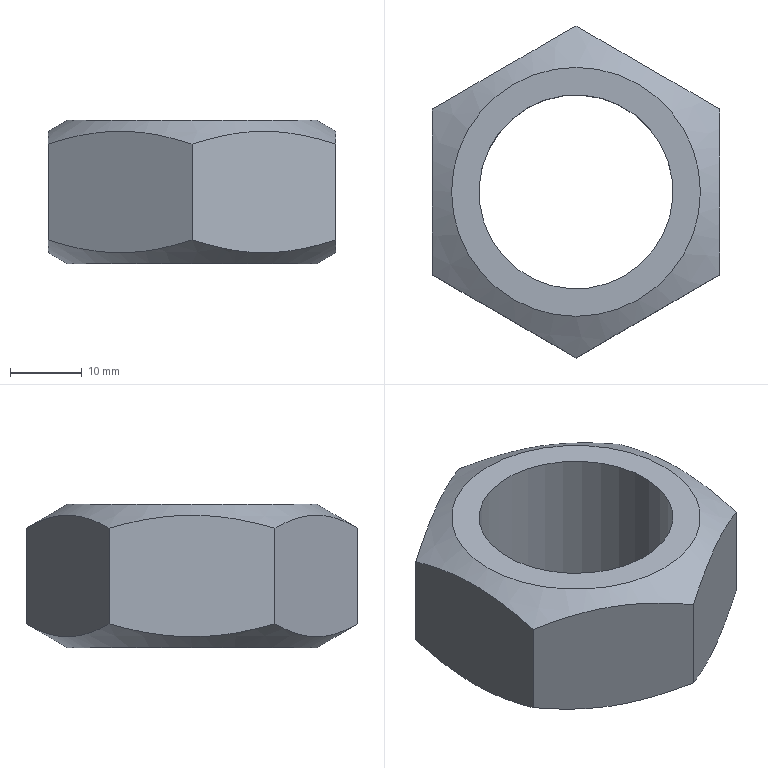Component | NX | NUT_M27 | 1 solid | 11 faces | volume 15223 mm3 | plane 8 | cone 2 | cylinder 1 | commonest cylinder face diameters 27 x1